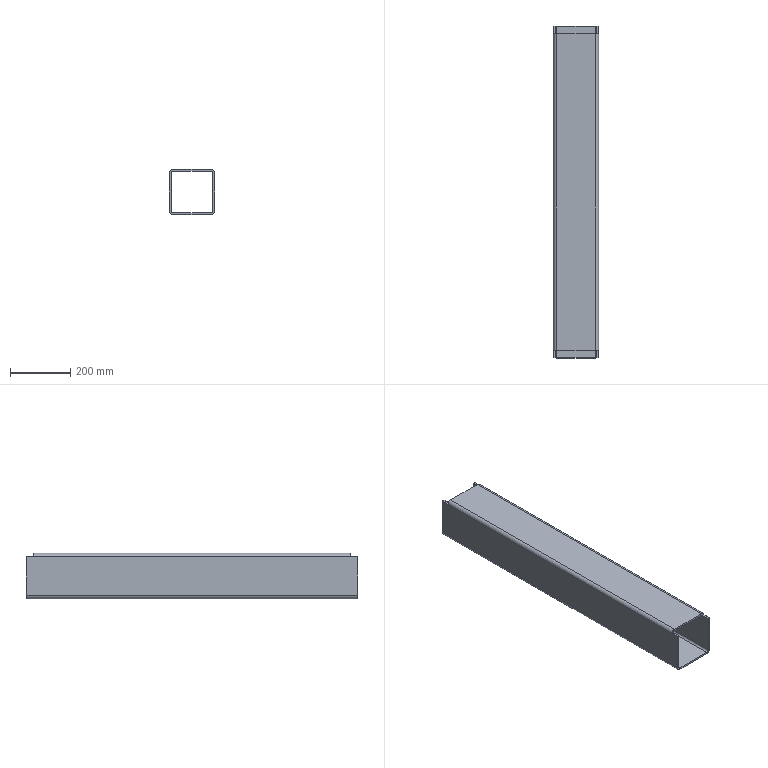Component | SolidWorks | Link1-13 | 1 solid | 24 faces | box 150 x 1100 x 150 mm | volume 3654550 mm3 | plane 16 | cylinder 8 | commonest cylinder face diameters 24 x4 12 x4 | material Plain Carbon Steel
build123d program:
from build123d import *

# Parameters (mm, degrees)
BOSS_EXTRUDE1_DEPTH = 1100
SKETCH3_W           = 150
SKETCH3_H           = 25
CUT_EXTRUDE1_DEPTH  = 10


with BuildPart() as part:
    # Sketch1 → Boss-Extrude1 (new body)
    with BuildSketch(Plane.XY):
        with BuildLine():
            Line((-63, -75), (63, -75))
            ThreePointArc((63, -75), (71.485, -71.485), (75, -63))
            Line((75, -63), (75, 63))
            ThreePointArc((75, 63), (71.485, 71.485), (63, 75))
            Line((63, 75), (-63, 75))
            ThreePointArc((-63, 75), (-71.485, 71.485), (-75, 63))
            Line((-75, 63), (-75, -63))
            ThreePointArc((-75, -63), (-71.485, -71.485), (-63, -75))
        make_face()
        with BuildLine():
            Line((-63, -69), (63, -69))
            ThreePointArc((63, -69), (67.243, -67.243), (69, -63))
            Line((69, -63), (69, 63))
            ThreePointArc((69, 63), (67.243, 67.243), (63, 69))
            Line((63, 69), (-63, 69))
            ThreePointArc((-63, 69), (-67.243, 67.243), (-69, 63))
            Line((-69, 63), (-69, -63))
            ThreePointArc((-69, -63), (-67.243, -67.243), (-63, -69))
        make_face(mode=Mode.SUBTRACT)
    extrude(amount=BOSS_EXTRUDE1_DEPTH)

    # Sketch3 → Cut-Extrude1 (cut)
    with BuildSketch(Plane(origin=(0, 75, 0), x_dir=(1, 0, 0), z_dir=(0, 1, 0))):
        with Locations((0, -12.5)):
            Rectangle(SKETCH3_W, SKETCH3_H)
        with Locations((0, -1087.5)):
            Rectangle(SKETCH3_W, SKETCH3_H)
    extrude(amount=-CUT_EXTRUDE1_DEPTH, mode=Mode.SUBTRACT)


solid = part.part

# Placed as in the assembly
solid = solid.moved(Location((157.801, 1721.323, 5500.973), (90, 0, 0)))
STEP:
#1=COLOUR_RGB('',0.7922,0.8196,0.9333);
#2=FILL_AREA_STYLE_COLOUR('',#1);
#3=FILL_AREA_STYLE('',(#2));
#4=SURFACE_STYLE_FILL_AREA(#3);
#5=SURFACE_SIDE_STYLE('',(#4));
#6=SURFACE_STYLE_USAGE(.BOTH.,#5);
#7=PRESENTATION_STYLE_ASSIGNMENT((#6));
#8=CARTESIAN_POINT('',(3.266,24.462,219.133));
#9=VERTEX_POINT('',#8);
#10=CARTESIAN_POINT('',(3.51,24.462,219.133));
#11=VERTEX_POINT('',#10);
#12=CARTESIAN_POINT('',(9.165,24.462,219.133));
#13=DIRECTION('',(1.,0.,0.));
#14=VECTOR('',#13,39.37);
#15=LINE('',#12,#14);
#16=EDGE_CURVE('',#9,#11,#15,.T.);
#17=ORIENTED_EDGE('',*,*,#16,.F.);
#18=CARTESIAN_POINT('',(3.26,24.462,219.054));
#19=VERTEX_POINT('',#18);
#20=CARTESIAN_POINT('',(3.732,24.462,219.054));
#21=DIRECTION('',(-0.,1.,0.));
#22=DIRECTION('',(-1.,0.,0.));
#23=AXIS2_PLACEMENT_3D('',#20,#21,#22);
#24=CIRCLE('',#23,0.4724);
#25=EDGE_CURVE('',#19,#9,#24,.T.);
#26=ORIENTED_EDGE('',*,*,#25,.F.);
#27=CARTESIAN_POINT('',(3.26,24.462,214.093));
#28=VERTEX_POINT('',#27);
#29=CARTESIAN_POINT('',(3.26,24.462,219.054));
#30=DIRECTION('',(-0.,0.,-1.));
#31=VECTOR('',#30,39.37);
#32=LINE('',#29,#31);
#33=EDGE_CURVE('',#19,#28,#32,.T.);
#34=ORIENTED_EDGE('',*,*,#33,.T.);
#35=CARTESIAN_POINT('',(3.732,24.462,213.621));
#36=VERTEX_POINT('',#35);
#37=CARTESIAN_POINT('',(3.732,24.462,214.093));
#38=DIRECTION('',(-0.,1.,0.));
#39=DIRECTION('',(-1.,0.,0.));
#40=AXIS2_PLACEMENT_3D('',#37,#38,#39);
#41=CIRCLE('',#40,0.4724);
#42=EDGE_CURVE('',#36,#28,#41,.T.);
#43=ORIENTED_EDGE('',*,*,#42,.F.);
#44=CARTESIAN_POINT('',(8.693,24.462,213.621));
#45=VERTEX_POINT('',#44);
#46=CARTESIAN_POINT('',(8.693,24.462,213.621));
#47=DIRECTION('',(-1.,-0.,-0.));
#48=VECTOR('',#47,39.37);
#49=LINE('',#46,#48);
#50=EDGE_CURVE('',#45,#36,#49,.T.);
#51=ORIENTED_EDGE('',*,*,#50,.F.);
#52=CARTESIAN_POINT('',(9.165,24.462,214.093));
#53=VERTEX_POINT('',#52);
#54=CARTESIAN_POINT('',(8.693,24.462,214.093));
#55=DIRECTION('',(-0.,1.,0.));
#56=DIRECTION('',(-1.,0.,0.));
#57=AXIS2_PLACEMENT_3D('',#54,#55,#56);
#58=CIRCLE('',#57,0.4724);
#59=EDGE_CURVE('',#53,#45,#58,.T.);
#60=ORIENTED_EDGE('',*,*,#59,.F.);
#61=CARTESIAN_POINT('',(9.165,24.462,219.054));
#62=VERTEX_POINT('',#61);
#63=CARTESIAN_POINT('',(9.165,24.462,214.093));
#64=DIRECTION('',(0.,-0.,1.));
#65=VECTOR('',#64,39.37);
#66=LINE('',#63,#65);
#67=EDGE_CURVE('',#53,#62,#66,.T.);
#68=ORIENTED_EDGE('',*,*,#67,.T.);
#69=CARTESIAN_POINT('',(9.159,24.462,219.133));
#70=VERTEX_POINT('',#69);
#71=CARTESIAN_POINT('',(8.693,24.462,219.054));
#72=DIRECTION('',(-0.,1.,0.));
#73=DIRECTION('',(-1.,0.,0.));
#74=AXIS2_PLACEMENT_3D('',#71,#72,#73);
#75=CIRCLE('',#74,0.4724);
#76=EDGE_CURVE('',#70,#62,#75,.T.);
#77=ORIENTED_EDGE('',*,*,#76,.F.);
#78=CARTESIAN_POINT('',(8.916,24.462,219.133));
#79=VERTEX_POINT('',#78);
#80=CARTESIAN_POINT('',(9.165,24.462,219.133));
#81=DIRECTION('',(1.,0.,0.));
#82=VECTOR('',#81,39.37);
#83=LINE('',#80,#82);
#84=EDGE_CURVE('',#79,#70,#83,.T.);
#85=ORIENTED_EDGE('',*,*,#84,.F.);
#86=CARTESIAN_POINT('',(8.929,24.462,219.054));
#87=VERTEX_POINT('',#86);
#88=CARTESIAN_POINT('',(8.693,24.462,219.054));
#89=DIRECTION('',(-0.,1.,0.));
#90=DIRECTION('',(-1.,0.,0.));
#91=AXIS2_PLACEMENT_3D('',#88,#89,#90);
#92=CIRCLE('',#91,0.2362);
#93=EDGE_CURVE('',#79,#87,#92,.T.);
#94=ORIENTED_EDGE('',*,*,#93,.T.);
#95=CARTESIAN_POINT('',(8.929,24.462,214.093));
#96=VERTEX_POINT('',#95);
#97=CARTESIAN_POINT('',(8.929,24.462,214.093));
#98=DIRECTION('',(0.,-0.,1.));
#99=VECTOR('',#98,39.37);
#100=LINE('',#97,#99);
#101=EDGE_CURVE('',#96,#87,#100,.T.);
#102=ORIENTED_EDGE('',*,*,#101,.F.);
#103=CARTESIAN_POINT('',(8.693,24.462,213.857));
#104=VERTEX_POINT('',#103);
#105=CARTESIAN_POINT('',(8.693,24.462,214.093));
#106=DIRECTION('',(-0.,1.,0.));
#107=DIRECTION('',(-1.,0.,0.));
#108=AXIS2_PLACEMENT_3D('',#105,#106,#107);
#109=CIRCLE('',#108,0.2362);
#110=EDGE_CURVE('',#96,#104,#109,.T.);
#111=ORIENTED_EDGE('',*,*,#110,.T.);
#112=CARTESIAN_POINT('',(3.732,24.462,213.857));
#113=VERTEX_POINT('',#112);
#114=CARTESIAN_POINT('',(8.693,24.462,213.857));
#115=DIRECTION('',(-1.,-0.,-0.));
#116=VECTOR('',#115,39.37);
#117=LINE('',#114,#116);
#118=EDGE_CURVE('',#104,#113,#117,.T.);
#119=ORIENTED_EDGE('',*,*,#118,.T.);
#120=CARTESIAN_POINT('',(3.496,24.462,214.093));
#121=VERTEX_POINT('',#120);
#122=CARTESIAN_POINT('',(3.732,24.462,214.093));
#123=DIRECTION('',(-0.,1.,0.));
#124=DIRECTION('',(-1.,0.,0.));
#125=AXIS2_PLACEMENT_3D('',#122,#123,#124);
#126=CIRCLE('',#125,0.2362);
#127=EDGE_CURVE('',#113,#121,#126,.T.);
#128=ORIENTED_EDGE('',*,*,#127,.T.);
#129=CARTESIAN_POINT('',(3.496,24.462,219.054));
#130=VERTEX_POINT('',#129);
#131=CARTESIAN_POINT('',(3.496,24.462,219.054));
#132=DIRECTION('',(-0.,0.,-1.));
#133=VECTOR('',#132,39.37);
#134=LINE('',#131,#133);
#135=EDGE_CURVE('',#130,#121,#134,.T.);
#136=ORIENTED_EDGE('',*,*,#135,.F.);
#137=CARTESIAN_POINT('',(3.732,24.462,219.054));
#138=DIRECTION('',(-0.,1.,0.));
#139=DIRECTION('',(-1.,0.,0.));
#140=AXIS2_PLACEMENT_3D('',#137,#138,#139);
#141=CIRCLE('',#140,0.2362);
#142=EDGE_CURVE('',#130,#11,#141,.T.);
#143=ORIENTED_EDGE('',*,*,#142,.T.);
#144=EDGE_LOOP('',(#17,#26,#34,#43,#51,#60,#68,#77,#85,#94,#102,#111,#119,#128,#136,#143));
#145=FACE_OUTER_BOUND('',#144,.T.);
#146=CARTESIAN_POINT('',(3.732,24.462,219.054));
#147=DIRECTION('',(-0.,1.,0.));
#148=DIRECTION('',(-1.,-0.,-0.));
#149=AXIS2_PLACEMENT_3D('',#146,#147,#148);
#150=PLANE('',#149);
#151=ADVANCED_FACE('',(#145),#150,.F.);
#152=CARTESIAN_POINT('',(9.159,67.769,219.133));
#153=VERTEX_POINT('',#152);
#154=CARTESIAN_POINT('',(8.916,67.769,219.133));
#155=VERTEX_POINT('',#154);
#156=CARTESIAN_POINT('',(9.165,67.769,219.133));
#157=DIRECTION('',(-1.,-0.,-0.));
#158=VECTOR('',#157,39.37);
#159=LINE('',#156,#158);
#160=EDGE_CURVE('',#153,#155,#159,.T.);
#161=ORIENTED_EDGE('',*,*,#160,.F.);
#162=CARTESIAN_POINT('',(9.165,67.769,219.054));
#163=VERTEX_POINT('',#162);
#164=CARTESIAN_POINT('',(8.693,67.769,219.054));
#165=DIRECTION('',(-0.,1.,0.));
#166=DIRECTION('',(-1.,0.,0.));
#167=AXIS2_PLACEMENT_3D('',#164,#165,#166);
#168=CIRCLE('',#167,0.4724);
#169=EDGE_CURVE('',#153,#163,#168,.T.);
#170=ORIENTED_EDGE('',*,*,#169,.T.);
#171=CARTESIAN_POINT('',(9.165,67.769,214.093));
#172=VERTEX_POINT('',#171);
#173=CARTESIAN_POINT('',(9.165,67.769,214.093));
#174=DIRECTION('',(0.,-0.,1.));
#175=VECTOR('',#174,39.37);
#176=LINE('',#173,#175);
#177=EDGE_CURVE('',#172,#163,#176,.T.);
#178=ORIENTED_EDGE('',*,*,#177,.F.);
#179=CARTESIAN_POINT('',(8.693,67.769,213.621));
#180=VERTEX_POINT('',#179);
#181=CARTESIAN_POINT('',(8.693,67.769,214.093));
#182=DIRECTION('',(-0.,1.,0.));
#183=DIRECTION('',(-1.,0.,0.));
#184=AXIS2_PLACEMENT_3D('',#181,#182,#183);
#185=CIRCLE('',#184,0.4724);
#186=EDGE_CURVE('',#172,#180,#185,.T.);
#187=ORIENTED_EDGE('',*,*,#186,.T.);
#188=CARTESIAN_POINT('',(3.732,67.769,213.621));
#189=VERTEX_POINT('',#188);
#190=CARTESIAN_POINT('',(8.693,67.769,213.621));
#191=DIRECTION('',(-1.,-0.,-0.));
#192=VECTOR('',#191,39.37);
#193=LINE('',#190,#192);
#194=EDGE_CURVE('',#180,#189,#193,.T.);
#195=ORIENTED_EDGE('',*,*,#194,.T.);
#196=CARTESIAN_POINT('',(3.26,67.769,214.093));
#197=VERTEX_POINT('',#196);
#198=CARTESIAN_POINT('',(3.732,67.769,214.093));
#199=DIRECTION('',(-0.,1.,0.));
#200=DIRECTION('',(-1.,0.,0.));
#201=AXIS2_PLACEMENT_3D('',#198,#199,#200);
#202=CIRCLE('',#201,0.4724);
#203=EDGE_CURVE('',#189,#197,#202,.T.);
#204=ORIENTED_EDGE('',*,*,#203,.T.);
#205=CARTESIAN_POINT('',(3.26,67.769,219.054));
#206=VERTEX_POINT('',#205);
#207=CARTESIAN_POINT('',(3.26,67.769,219.054));
#208=DIRECTION('',(-0.,0.,-1.));
#209=VECTOR('',#208,39.37);
#210=LINE('',#207,#209);
#211=EDGE_CURVE('',#206,#197,#210,.T.);
#212=ORIENTED_EDGE('',*,*,#211,.F.);
#213=CARTESIAN_POINT('',(3.266,67.769,219.133));
#214=VERTEX_POINT('',#213);
#215=CARTESIAN_POINT('',(3.732,67.769,219.054));
#216=DIRECTION('',(-0.,1.,0.));
#217=DIRECTION('',(-1.,0.,0.));
#218=AXIS2_PLACEMENT_3D('',#215,#216,#217);
#219=CIRCLE('',#218,0.4724);
#220=EDGE_CURVE('',#206,#214,#219,.T.);
#221=ORIENTED_EDGE('',*,*,#220,.T.);
#222=CARTESIAN_POINT('',(3.51,67.769,219.133));
#223=VERTEX_POINT('',#222);
#224=CARTESIAN_POINT('',(9.165,67.769,219.133));
#225=DIRECTION('',(-1.,-0.,-0.));
#226=VECTOR('',#225,39.37);
#227=LINE('',#224,#226);
#228=EDGE_CURVE('',#223,#214,#227,.T.);
#229=ORIENTED_EDGE('',*,*,#228,.F.);
#230=CARTESIAN_POINT('',(3.496,67.769,219.054));
#231=VERTEX_POINT('',#230);
#232=CARTESIAN_POINT('',(3.732,67.769,219.054));
#233=DIRECTION('',(-0.,1.,0.));
#234=DIRECTION('',(-1.,0.,0.));
#235=AXIS2_PLACEMENT_3D('',#232,#233,#234);
#236=CIRCLE('',#235,0.2362);
#237=EDGE_CURVE('',#231,#223,#236,.T.);
#238=ORIENTED_EDGE('',*,*,#237,.F.);
#239=CARTESIAN_POINT('',(3.496,67.769,214.093));
#240=VERTEX_POINT('',#239);
#241=CARTESIAN_POINT('',(3.496,67.769,219.054));
#242=DIRECTION('',(-0.,0.,-1.));
#243=VECTOR('',#242,39.37);
#244=LINE('',#241,#243);
#245=EDGE_CURVE('',#231,#240,#244,.T.);
#246=ORIENTED_EDGE('',*,*,#245,.T.);
#247=CARTESIAN_POINT('',(3.732,67.769,213.857));
#248=VERTEX_POINT('',#247);
#249=CARTESIAN_POINT('',(3.732,67.769,214.093));
#250=DIRECTION('',(-0.,1.,0.));
#251=DIRECTION('',(-1.,0.,0.));
#252=AXIS2_PLACEMENT_3D('',#249,#250,#251);
#253=CIRCLE('',#252,0.2362);
#254=EDGE_CURVE('',#248,#240,#253,.T.);
#255=ORIENTED_EDGE('',*,*,#254,.F.);
#256=CARTESIAN_POINT('',(8.693,67.769,213.857));
#257=VERTEX_POINT('',#256);
#258=CARTESIAN_POINT('',(8.693,67.769,213.857));
#259=DIRECTION('',(-1.,-0.,-0.));
#260=VECTOR('',#259,39.37);
#261=LINE('',#258,#260);
#262=EDGE_CURVE('',#257,#248,#261,.T.);
#263=ORIENTED_EDGE('',*,*,#262,.F.);
#264=CARTESIAN_POINT('',(8.929,67.769,214.093));
#265=VERTEX_POINT('',#264);
#266=CARTESIAN_POINT('',(8.693,67.769,214.093));
#267=DIRECTION('',(-0.,1.,0.));
#268=DIRECTION('',(-1.,0.,0.));
#269=AXIS2_PLACEMENT_3D('',#266,#267,#268);
#270=CIRCLE('',#269,0.2362);
#271=EDGE_CURVE('',#265,#257,#270,.T.);
#272=ORIENTED_EDGE('',*,*,#271,.F.);
#273=CARTESIAN_POINT('',(8.929,67.769,219.054));
#274=VERTEX_POINT('',#273);
#275=CARTESIAN_POINT('',(8.929,67.769,214.093));
#276=DIRECTION('',(0.,-0.,1.));
#277=VECTOR('',#276,39.37);
#278=LINE('',#275,#277);
#279=EDGE_CURVE('',#265,#274,#278,.T.);
#280=ORIENTED_EDGE('',*,*,#279,.T.);
#281=CARTESIAN_POINT('',(8.693,67.769,219.054));
#282=DIRECTION('',(-0.,1.,0.));
#283=DIRECTION('',(-1.,0.,0.));
#284=AXIS2_PLACEMENT_3D('',#281,#282,#283);
#285=CIRCLE('',#284,0.2362);
#286=EDGE_CURVE('',#155,#274,#285,.T.);
#287=ORIENTED_EDGE('',*,*,#286,.F.);
#288=EDGE_LOOP('',(#161,#170,#178,#187,#195,#204,#212,#221,#229,#238,#246,#255,#263,#272,#280,#287));
#289=FACE_OUTER_BOUND('',#288,.T.);
#290=CARTESIAN_POINT('',(3.732,67.769,219.054));
#291=DIRECTION('',(-0.,1.,0.));
#292=DIRECTION('',(-1.,-0.,-0.));
#293=AXIS2_PLACEMENT_3D('',#290,#291,#292);
#294=PLANE('',#293);
#295=ADVANCED_FACE('',(#289),#294,.T.);
#296=CARTESIAN_POINT('',(3.266,25.446,219.133));
#297=VERTEX_POINT('',#296);
#298=CARTESIAN_POINT('',(3.266,67.769,219.133));
#299=DIRECTION('',(0.,-1.,-0.));
#300=VECTOR('',#299,39.37);
#301=LINE('',#298,#300);
#302=EDGE_CURVE('',#297,#9,#301,.T.);
#303=ORIENTED_EDGE('',*,*,#302,.F.);
#304=CARTESIAN_POINT('',(3.732,25.446,219.527));
#305=VERTEX_POINT('',#304);
#306=CARTESIAN_POINT('',(3.732,25.446,219.054));
#307=DIRECTION('',(-0.,1.,0.));
#308=DIRECTION('',(-1.,0.,0.));
#309=AXIS2_PLACEMENT_3D('',#306,#307,#308);
#310=CIRCLE('',#309,0.4724);
#311=EDGE_CURVE('',#297,#305,#310,.T.);
#312=ORIENTED_EDGE('',*,*,#311,.T.);
#313=CARTESIAN_POINT('',(3.732,66.784,219.527));
#314=VERTEX_POINT('',#313);
#315=CARTESIAN_POINT('',(3.732,67.769,219.527));
#316=DIRECTION('',(0.,-1.,-0.));
#317=VECTOR('',#316,39.37);
#318=LINE('',#315,#317);
#319=EDGE_CURVE('',#314,#305,#318,.T.);
#320=ORIENTED_EDGE('',*,*,#319,.F.);
#321=CARTESIAN_POINT('',(3.266,66.784,219.133));
#322=VERTEX_POINT('',#321);
#323=CARTESIAN_POINT('',(3.732,66.784,219.054));
#324=DIRECTION('',(0.,-1.,-0.));
#325=DIRECTION('',(1.,0.,0.));
#326=AXIS2_PLACEMENT_3D('',#323,#324,#325);
#327=CIRCLE('',#326,0.4724);
#328=EDGE_CURVE('',#314,#322,#327,.T.);
#329=ORIENTED_EDGE('',*,*,#328,.T.);
#330=CARTESIAN_POINT('',(3.266,67.769,219.133));
#331=DIRECTION('',(-0.,1.,0.));
#332=VECTOR('',#331,39.37);
#333=LINE('',#330,#332);
#334=EDGE_CURVE('',#322,#214,#333,.T.);
#335=ORIENTED_EDGE('',*,*,#334,.T.);
#336=ORIENTED_EDGE('',*,*,#220,.F.);
#337=CARTESIAN_POINT('',(3.26,67.769,219.054));
#338=DIRECTION('',(0.,-1.,-0.));
#339=VECTOR('',#338,39.37);
#340=LINE('',#337,#339);
#341=EDGE_CURVE('',#206,#19,#340,.T.);
#342=ORIENTED_EDGE('',*,*,#341,.T.);
#343=ORIENTED_EDGE('',*,*,#25,.T.);
#344=EDGE_LOOP('',(#303,#312,#320,#329,#335,#336,#342,#343));
#345=FACE_OUTER_BOUND('',#344,.T.);
#346=CARTESIAN_POINT('',(3.732,67.769,219.054));
#347=DIRECTION('',(0.,-1.,-0.));
#348=DIRECTION('',(1.,0.,0.));
#349=AXIS2_PLACEMENT_3D('',#346,#347,#348);
#350=CYLINDRICAL_SURFACE('',#349,0.4724);
#351=ADVANCED_FACE('',(#345),#350,.T.);
#352=ORIENTED_EDGE('',*,*,#319,.T.);
#353=CARTESIAN_POINT('',(8.693,25.446,219.527));
#354=VERTEX_POINT('',#353);
#355=CARTESIAN_POINT('',(9.165,25.446,219.527));
#356=DIRECTION('',(-1.,-0.,-0.));
#357=VECTOR('',#356,39.37);
#358=LINE('',#355,#357);
#359=EDGE_CURVE('',#354,#305,#358,.T.);
#360=ORIENTED_EDGE('',*,*,#359,.F.);
#361=CARTESIAN_POINT('',(8.693,66.784,219.527));
#362=VERTEX_POINT('',#361);
#363=CARTESIAN_POINT('',(8.693,67.769,219.527));
#364=DIRECTION('',(0.,-1.,-0.));
#365=VECTOR('',#364,39.37);
#366=LINE('',#363,#365);
#367=EDGE_CURVE('',#362,#354,#366,.T.);
#368=ORIENTED_EDGE('',*,*,#367,.F.);
#369=CARTESIAN_POINT('',(9.165,66.784,219.527));
#370=DIRECTION('',(1.,0.,0.));
#371=VECTOR('',#370,39.37);
#372=LINE('',#369,#371);
#373=EDGE_CURVE('',#314,#362,#372,.T.);
#374=ORIENTED_EDGE('',*,*,#373,.F.);
#375=EDGE_LOOP('',(#352,#360,#368,#374));
#376=FACE_OUTER_BOUND('',#375,.T.);
#377=CARTESIAN_POINT('',(3.732,67.769,219.527));
#378=DIRECTION('',(-0.,0.,-1.));
#379=DIRECTION('',(0.,-1.,-0.));
#380=AXIS2_PLACEMENT_3D('',#377,#378,#379);
#381=PLANE('',#380);
#382=ADVANCED_FACE('',(#376),#381,.F.);
#383=ORIENTED_EDGE('',*,*,#367,.T.);
#384=CARTESIAN_POINT('',(9.159,25.446,219.133));
#385=VERTEX_POINT('',#384);
#386=CARTESIAN_POINT('',(8.693,25.446,219.054));
#387=DIRECTION('',(-0.,1.,0.));
#388=DIRECTION('',(-1.,0.,0.));
#389=AXIS2_PLACEMENT_3D('',#386,#387,#388);
#390=CIRCLE('',#389,0.4724);
#391=EDGE_CURVE('',#354,#385,#390,.T.);
#392=ORIENTED_EDGE('',*,*,#391,.T.);
#393=CARTESIAN_POINT('',(9.159,67.769,219.133));
#394=DIRECTION('',(-0.,1.,0.));
#395=VECTOR('',#394,39.37);
#396=LINE('',#393,#395);
#397=EDGE_CURVE('',#70,#385,#396,.T.);
#398=ORIENTED_EDGE('',*,*,#397,.F.);
#399=ORIENTED_EDGE('',*,*,#76,.T.);
#400=CARTESIAN_POINT('',(9.165,67.769,219.054));
#401=DIRECTION('',(0.,-1.,-0.));
#402=VECTOR('',#401,39.37);
#403=LINE('',#400,#402);
#404=EDGE_CURVE('',#163,#62,#403,.T.);
#405=ORIENTED_EDGE('',*,*,#404,.F.);
#406=ORIENTED_EDGE('',*,*,#169,.F.);
#407=CARTESIAN_POINT('',(9.159,66.784,219.133));
#408=VERTEX_POINT('',#407);
#409=CARTESIAN_POINT('',(9.159,67.769,219.133));
#410=DIRECTION('',(0.,-1.,-0.));
#411=VECTOR('',#410,39.37);
#412=LINE('',#409,#411);
#413=EDGE_CURVE('',#153,#408,#412,.T.);
#414=ORIENTED_EDGE('',*,*,#413,.T.);
#415=CARTESIAN_POINT('',(8.693,66.784,219.054));
#416=DIRECTION('',(0.,-1.,-0.));
#417=DIRECTION('',(1.,0.,0.));
#418=AXIS2_PLACEMENT_3D('',#415,#416,#417);
#419=CIRCLE('',#418,0.4724);
#420=EDGE_CURVE('',#408,#362,#419,.T.);
#421=ORIENTED_EDGE('',*,*,#420,.T.);
#422=EDGE_LOOP('',(#383,#392,#398,#399,#405,#406,#414,#421));
#423=FACE_OUTER_BOUND('',#422,.T.);
#424=CARTESIAN_POINT('',(8.693,67.769,219.054));
#425=DIRECTION('',(0.,-1.,-0.));
#426=DIRECTION('',(1.,0.,0.));
#427=AXIS2_PLACEMENT_3D('',#424,#425,#426);
#428=CYLINDRICAL_SURFACE('',#427,0.4724);
#429=ADVANCED_FACE('',(#423),#428,.T.);
#430=ORIENTED_EDGE('',*,*,#67,.F.);
#431=CARTESIAN_POINT('',(9.165,67.769,214.093));
#432=DIRECTION('',(0.,-1.,-0.));
#433=VECTOR('',#432,39.37);
#434=LINE('',#431,#433);
#435=EDGE_CURVE('',#172,#53,#434,.T.);
#436=ORIENTED_EDGE('',*,*,#435,.F.);
#437=ORIENTED_EDGE('',*,*,#177,.T.);
#438=ORIENTED_EDGE('',*,*,#404,.T.);
#439=EDGE_LOOP('',(#430,#436,#437,#438));
#440=FACE_OUTER_BOUND('',#439,.T.);
#441=CARTESIAN_POINT('',(9.165,67.769,214.093));
#442=DIRECTION('',(1.,0.,0.));
#443=DIRECTION('',(-0.,1.,0.));
#444=AXIS2_PLACEMENT_3D('',#441,#442,#443);
#445=PLANE('',#444);
#446=ADVANCED_FACE('',(#440),#445,.T.);
#447=ORIENTED_EDGE('',*,*,#59,.T.);
#448=CARTESIAN_POINT('',(8.693,67.769,213.621));
#449=DIRECTION('',(0.,-1.,-0.));
#450=VECTOR('',#449,39.37);
#451=LINE('',#448,#450);
#452=EDGE_CURVE('',#180,#45,#451,.T.);
#453=ORIENTED_EDGE('',*,*,#452,.F.);
#454=ORIENTED_EDGE('',*,*,#186,.F.);
#455=ORIENTED_EDGE('',*,*,#435,.T.);
#456=EDGE_LOOP('',(#447,#453,#454,#455));
#457=FACE_OUTER_BOUND('',#456,.T.);
#458=CARTESIAN_POINT('',(8.693,67.769,214.093));
#459=DIRECTION('',(0.,-1.,-0.));
#460=DIRECTION('',(1.,0.,0.));
#461=AXIS2_PLACEMENT_3D('',#458,#459,#460);
#462=CYLINDRICAL_SURFACE('',#461,0.4724);
#463=ADVANCED_FACE('',(#457),#462,.T.);
#464=ORIENTED_EDGE('',*,*,#50,.T.);
#465=CARTESIAN_POINT('',(3.732,67.769,213.621));
#466=DIRECTION('',(0.,-1.,-0.));
#467=VECTOR('',#466,39.37);
#468=LINE('',#465,#467);
#469=EDGE_CURVE('',#189,#36,#468,.T.);
#470=ORIENTED_EDGE('',*,*,#469,.F.);
#471=ORIENTED_EDGE('',*,*,#194,.F.);
#472=ORIENTED_EDGE('',*,*,#452,.T.);
#473=EDGE_LOOP('',(#464,#470,#471,#472));
#474=FACE_OUTER_BOUND('',#473,.T.);
#475=CARTESIAN_POINT('',(8.693,67.769,213.621));
#476=DIRECTION('',(0.,-0.,1.));
#477=DIRECTION('',(-0.,1.,0.));
#478=AXIS2_PLACEMENT_3D('',#475,#476,#477);
#479=PLANE('',#478);
#480=ADVANCED_FACE('',(#474),#479,.F.);
#481=ORIENTED_EDGE('',*,*,#42,.T.);
#482=CARTESIAN_POINT('',(3.26,67.769,214.093));
#483=DIRECTION('',(0.,-1.,-0.));
#484=VECTOR('',#483,39.37);
#485=LINE('',#482,#484);
#486=EDGE_CURVE('',#197,#28,#485,.T.);
#487=ORIENTED_EDGE('',*,*,#486,.F.);
#488=ORIENTED_EDGE('',*,*,#203,.F.);
#489=ORIENTED_EDGE('',*,*,#469,.T.);
#490=EDGE_LOOP('',(#481,#487,#488,#489));
#491=FACE_OUTER_BOUND('',#490,.T.);
#492=CARTESIAN_POINT('',(3.732,67.769,214.093));
#493=DIRECTION('',(0.,-1.,-0.));
#494=DIRECTION('',(1.,0.,0.));
#495=AXIS2_PLACEMENT_3D('',#492,#493,#494);
#496=CYLINDRICAL_SURFACE('',#495,0.4724);
#497=ADVANCED_FACE('',(#491),#496,.T.);
#498=ORIENTED_EDGE('',*,*,#33,.F.);
#499=ORIENTED_EDGE('',*,*,#341,.F.);
#500=ORIENTED_EDGE('',*,*,#211,.T.);
#501=ORIENTED_EDGE('',*,*,#486,.T.);
#502=EDGE_LOOP('',(#498,#499,#500,#501));
#503=FACE_OUTER_BOUND('',#502,.T.);
#504=CARTESIAN_POINT('',(3.26,67.769,219.054));
#505=DIRECTION('',(-1.,-0.,-0.));
#506=DIRECTION('',(0.,-1.,-0.));
#507=AXIS2_PLACEMENT_3D('',#504,#505,#506);
#508=PLANE('',#507);
#509=ADVANCED_FACE('',(#503),#508,.T.);
#510=ORIENTED_EDGE('',*,*,#110,.F.);
#511=CARTESIAN_POINT('',(8.929,67.769,214.093));
#512=DIRECTION('',(0.,-1.,-0.));
#513=VECTOR('',#512,39.37);
#514=LINE('',#511,#513);
#515=EDGE_CURVE('',#265,#96,#514,.T.);
#516=ORIENTED_EDGE('',*,*,#515,.F.);
#517=ORIENTED_EDGE('',*,*,#271,.T.);
#518=CARTESIAN_POINT('',(8.693,67.769,213.857));
#519=DIRECTION('',(0.,-1.,-0.));
#520=VECTOR('',#519,39.37);
#521=LINE('',#518,#520);
#522=EDGE_CURVE('',#257,#104,#521,.T.);
#523=ORIENTED_EDGE('',*,*,#522,.T.);
#524=EDGE_LOOP('',(#510,#516,#517,#523));
#525=FACE_OUTER_BOUND('',#524,.T.);
#526=CARTESIAN_POINT('',(8.693,67.769,214.093));
#527=DIRECTION('',(0.,-1.,-0.));
#528=DIRECTION('',(1.,0.,0.));
#529=AXIS2_PLACEMENT_3D('',#526,#527,#528);
#530=CYLINDRICAL_SURFACE('',#529,0.2362);
#531=ADVANCED_FACE('',(#525),#530,.F.);
#532=ORIENTED_EDGE('',*,*,#118,.F.);
#533=ORIENTED_EDGE('',*,*,#522,.F.);
#534=ORIENTED_EDGE('',*,*,#262,.T.);
#535=CARTESIAN_POINT('',(3.732,67.769,213.857));
#536=DIRECTION('',(0.,-1.,-0.));
#537=VECTOR('',#536,39.37);
#538=LINE('',#535,#537);
#539=EDGE_CURVE('',#248,#113,#538,.T.);
#540=ORIENTED_EDGE('',*,*,#539,.T.);
#541=EDGE_LOOP('',(#532,#533,#534,#540));
#542=FACE_OUTER_BOUND('',#541,.T.);
#543=CARTESIAN_POINT('',(8.693,67.769,213.857));
#544=DIRECTION('',(0.,-0.,1.));
#545=DIRECTION('',(-0.,1.,0.));
#546=AXIS2_PLACEMENT_3D('',#543,#544,#545);
#547=PLANE('',#546);
#548=ADVANCED_FACE('',(#542),#547,.T.);
#549=ORIENTED_EDGE('',*,*,#127,.F.);
#550=ORIENTED_EDGE('',*,*,#539,.F.);
#551=ORIENTED_EDGE('',*,*,#254,.T.);
#552=CARTESIAN_POINT('',(3.496,67.769,214.093));
#553=DIRECTION('',(0.,-1.,-0.));
#554=VECTOR('',#553,39.37);
#555=LINE('',#552,#554);
#556=EDGE_CURVE('',#240,#121,#555,.T.);
#557=ORIENTED_EDGE('',*,*,#556,.T.);
#558=EDGE_LOOP('',(#549,#550,#551,#557));
#559=FACE_OUTER_BOUND('',#558,.T.);
#560=CARTESIAN_POINT('',(3.732,67.769,214.093));
#561=DIRECTION('',(0.,-1.,-0.));
#562=DIRECTION('',(1.,0.,0.));
#563=AXIS2_PLACEMENT_3D('',#560,#561,#562);
#564=CYLINDRICAL_SURFACE('',#563,0.2362);
#565=ADVANCED_FACE('',(#559),#564,.F.);
#566=ORIENTED_EDGE('',*,*,#135,.T.);
#567=ORIENTED_EDGE('',*,*,#556,.F.);
#568=ORIENTED_EDGE('',*,*,#245,.F.);
#569=CARTESIAN_POINT('',(3.496,67.769,219.054));
#570=DIRECTION('',(0.,-1.,-0.));
#571=VECTOR('',#570,39.37);
#572=LINE('',#569,#571);
#573=EDGE_CURVE('',#231,#130,#572,.T.);
#574=ORIENTED_EDGE('',*,*,#573,.T.);
#575=EDGE_LOOP('',(#566,#567,#568,#574));
#576=FACE_OUTER_BOUND('',#575,.T.);
#577=CARTESIAN_POINT('',(3.496,67.769,219.054));
#578=DIRECTION('',(-1.,-0.,-0.));
#579=DIRECTION('',(0.,-1.,-0.));
#580=AXIS2_PLACEMENT_3D('',#577,#578,#579);
#581=PLANE('',#580);
#582=ADVANCED_FACE('',(#576),#581,.F.);
#583=CARTESIAN_POINT('',(3.51,25.446,219.133));
#584=VERTEX_POINT('',#583);
#585=CARTESIAN_POINT('',(3.732,25.446,219.29));
#586=VERTEX_POINT('',#585);
#587=CARTESIAN_POINT('',(3.732,25.446,219.054));
#588=DIRECTION('',(-0.,1.,0.));
#589=DIRECTION('',(-1.,0.,0.));
#590=AXIS2_PLACEMENT_3D('',#587,#588,#589);
#591=CIRCLE('',#590,0.2362);
#592=EDGE_CURVE('',#584,#586,#591,.T.);
#593=ORIENTED_EDGE('',*,*,#592,.F.);
#594=CARTESIAN_POINT('',(3.51,67.769,219.133));
#595=DIRECTION('',(0.,-1.,-0.));
#596=VECTOR('',#595,39.37);
#597=LINE('',#594,#596);
#598=EDGE_CURVE('',#584,#11,#597,.T.);
#599=ORIENTED_EDGE('',*,*,#598,.T.);
#600=ORIENTED_EDGE('',*,*,#142,.F.);
#601=ORIENTED_EDGE('',*,*,#573,.F.);
#602=ORIENTED_EDGE('',*,*,#237,.T.);
#603=CARTESIAN_POINT('',(3.51,66.784,219.133));
#604=VERTEX_POINT('',#603);
#605=CARTESIAN_POINT('',(3.51,67.769,219.133));
#606=DIRECTION('',(-0.,1.,0.));
#607=VECTOR('',#606,39.37);
#608=LINE('',#605,#607);
#609=EDGE_CURVE('',#604,#223,#608,.T.);
#610=ORIENTED_EDGE('',*,*,#609,.F.);
#611=CARTESIAN_POINT('',(3.732,66.784,219.29));
#612=VERTEX_POINT('',#611);
#613=CARTESIAN_POINT('',(3.732,66.784,219.054));
#614=DIRECTION('',(0.,-1.,-0.));
#615=DIRECTION('',(1.,0.,0.));
#616=AXIS2_PLACEMENT_3D('',#613,#614,#615);
#617=CIRCLE('',#616,0.2362);
#618=EDGE_CURVE('',#612,#604,#617,.T.);
#619=ORIENTED_EDGE('',*,*,#618,.F.);
#620=CARTESIAN_POINT('',(3.732,67.769,219.29));
#621=DIRECTION('',(0.,-1.,-0.));
#622=VECTOR('',#621,39.37);
#623=LINE('',#620,#622);
#624=EDGE_CURVE('',#612,#586,#623,.T.);
#625=ORIENTED_EDGE('',*,*,#624,.T.);
#626=EDGE_LOOP('',(#593,#599,#600,#601,#602,#610,#619,#625));
#627=FACE_OUTER_BOUND('',#626,.T.);
#628=CARTESIAN_POINT('',(3.732,67.769,219.054));
#629=DIRECTION('',(0.,-1.,-0.));
#630=DIRECTION('',(1.,0.,0.));
#631=AXIS2_PLACEMENT_3D('',#628,#629,#630);
#632=CYLINDRICAL_SURFACE('',#631,0.2362);
#633=ADVANCED_FACE('',(#627),#632,.F.);
#634=CARTESIAN_POINT('',(8.693,25.446,219.29));
#635=VERTEX_POINT('',#634);
#636=CARTESIAN_POINT('',(3.732,25.446,219.29));
#637=DIRECTION('',(1.,0.,0.));
#638=VECTOR('',#637,39.37);
#639=LINE('',#636,#638);
#640=EDGE_CURVE('',#586,#635,#639,.T.);
#641=ORIENTED_EDGE('',*,*,#640,.F.);
#642=ORIENTED_EDGE('',*,*,#624,.F.);
#643=CARTESIAN_POINT('',(8.693,66.784,219.29));
#644=VERTEX_POINT('',#643);
#645=CARTESIAN_POINT('',(3.732,66.784,219.29));
#646=DIRECTION('',(-1.,-0.,-0.));
#647=VECTOR('',#646,39.37);
#648=LINE('',#645,#647);
#649=EDGE_CURVE('',#644,#612,#648,.T.);
#650=ORIENTED_EDGE('',*,*,#649,.F.);
#651=CARTESIAN_POINT('',(8.693,67.769,219.29));
#652=DIRECTION('',(0.,-1.,-0.));
#653=VECTOR('',#652,39.37);
#654=LINE('',#651,#653);
#655=EDGE_CURVE('',#644,#635,#654,.T.);
#656=ORIENTED_EDGE('',*,*,#655,.T.);
#657=EDGE_LOOP('',(#641,#642,#650,#656));
#658=FACE_OUTER_BOUND('',#657,.T.);
#659=CARTESIAN_POINT('',(3.732,67.769,219.29));
#660=DIRECTION('',(-0.,0.,-1.));
#661=DIRECTION('',(0.,-1.,-0.));
#662=AXIS2_PLACEMENT_3D('',#659,#660,#661);
#663=PLANE('',#662);
#664=ADVANCED_FACE('',(#658),#663,.T.);
#665=CARTESIAN_POINT('',(8.916,25.446,219.133));
#666=VERTEX_POINT('',#665);
#667=CARTESIAN_POINT('',(8.693,25.446,219.054));
#668=DIRECTION('',(-0.,1.,0.));
#669=DIRECTION('',(-1.,0.,0.));
#670=AXIS2_PLACEMENT_3D('',#667,#668,#669);
#671=CIRCLE('',#670,0.2362);
#672=EDGE_CURVE('',#635,#666,#671,.T.);
#673=ORIENTED_EDGE('',*,*,#672,.F.);
#674=ORIENTED_EDGE('',*,*,#655,.F.);
#675=CARTESIAN_POINT('',(8.916,66.784,219.133));
#676=VERTEX_POINT('',#675);
#677=CARTESIAN_POINT('',(8.693,66.784,219.054));
#678=DIRECTION('',(0.,-1.,-0.));
#679=DIRECTION('',(1.,0.,0.));
#680=AXIS2_PLACEMENT_3D('',#677,#678,#679);
#681=CIRCLE('',#680,0.2362);
#682=EDGE_CURVE('',#676,#644,#681,.T.);
#683=ORIENTED_EDGE('',*,*,#682,.F.);
#684=CARTESIAN_POINT('',(8.916,67.769,219.133));
#685=DIRECTION('',(0.,-1.,-0.));
#686=VECTOR('',#685,39.37);
#687=LINE('',#684,#686);
#688=EDGE_CURVE('',#155,#676,#687,.T.);
#689=ORIENTED_EDGE('',*,*,#688,.F.);
#690=ORIENTED_EDGE('',*,*,#286,.T.);
#691=CARTESIAN_POINT('',(8.929,67.769,219.054));
#692=DIRECTION('',(0.,-1.,-0.));
#693=VECTOR('',#692,39.37);
#694=LINE('',#691,#693);
#695=EDGE_CURVE('',#274,#87,#694,.T.);
#696=ORIENTED_EDGE('',*,*,#695,.T.);
#697=ORIENTED_EDGE('',*,*,#93,.F.);
#698=CARTESIAN_POINT('',(8.916,67.769,219.133));
#699=DIRECTION('',(-0.,1.,0.));
#700=VECTOR('',#699,39.37);
#701=LINE('',#698,#700);
#702=EDGE_CURVE('',#79,#666,#701,.T.);
#703=ORIENTED_EDGE('',*,*,#702,.T.);
#704=EDGE_LOOP('',(#673,#674,#683,#689,#690,#696,#697,#703));
#705=FACE_OUTER_BOUND('',#704,.T.);
#706=CARTESIAN_POINT('',(8.693,67.769,219.054));
#707=DIRECTION('',(0.,-1.,-0.));
#708=DIRECTION('',(1.,0.,0.));
#709=AXIS2_PLACEMENT_3D('',#706,#707,#708);
#710=CYLINDRICAL_SURFACE('',#709,0.2362);
#711=ADVANCED_FACE('',(#705),#710,.F.);
#712=ORIENTED_EDGE('',*,*,#101,.T.);
#713=ORIENTED_EDGE('',*,*,#695,.F.);
#714=ORIENTED_EDGE('',*,*,#279,.F.);
#715=ORIENTED_EDGE('',*,*,#515,.T.);
#716=EDGE_LOOP('',(#712,#713,#714,#715));
#717=FACE_OUTER_BOUND('',#716,.T.);
#718=CARTESIAN_POINT('',(8.929,67.769,214.093));
#719=DIRECTION('',(1.,0.,0.));
#720=DIRECTION('',(-0.,1.,0.));
#721=AXIS2_PLACEMENT_3D('',#718,#719,#720);
#722=PLANE('',#721);
#723=ADVANCED_FACE('',(#717),#722,.F.);
#724=ORIENTED_EDGE('',*,*,#373,.T.);
#725=ORIENTED_EDGE('',*,*,#420,.F.);
#726=CARTESIAN_POINT('',(9.165,66.784,219.133));
#727=DIRECTION('',(1.,0.,0.));
#728=VECTOR('',#727,39.37);
#729=LINE('',#726,#728);
#730=EDGE_CURVE('',#676,#408,#729,.T.);
#731=ORIENTED_EDGE('',*,*,#730,.F.);
#732=ORIENTED_EDGE('',*,*,#682,.T.);
#733=ORIENTED_EDGE('',*,*,#649,.T.);
#734=ORIENTED_EDGE('',*,*,#618,.T.);
#735=CARTESIAN_POINT('',(9.165,66.784,219.133));
#736=DIRECTION('',(1.,0.,0.));
#737=VECTOR('',#736,39.37);
#738=LINE('',#735,#737);
#739=EDGE_CURVE('',#322,#604,#738,.T.);
#740=ORIENTED_EDGE('',*,*,#739,.F.);
#741=ORIENTED_EDGE('',*,*,#328,.F.);
#742=EDGE_LOOP('',(#724,#725,#731,#732,#733,#734,#740,#741));
#743=FACE_OUTER_BOUND('',#742,.T.);
#744=CARTESIAN_POINT('',(9.165,66.784,219.133));
#745=DIRECTION('',(0.,-1.,-0.));
#746=DIRECTION('',(1.,0.,0.));
#747=AXIS2_PLACEMENT_3D('',#744,#745,#746);
#748=PLANE('',#747);
#749=ADVANCED_FACE('',(#743),#748,.F.);
#750=ORIENTED_EDGE('',*,*,#739,.T.);
#751=ORIENTED_EDGE('',*,*,#609,.T.);
#752=ORIENTED_EDGE('',*,*,#228,.T.);
#753=ORIENTED_EDGE('',*,*,#334,.F.);
#754=EDGE_LOOP('',(#750,#751,#752,#753));
#755=FACE_OUTER_BOUND('',#754,.T.);
#756=CARTESIAN_POINT('',(6.213,24.462,219.133));
#757=DIRECTION('',(-0.,0.,-1.));
#758=DIRECTION('',(0.,-1.,-0.));
#759=AXIS2_PLACEMENT_3D('',#756,#757,#758);
#760=PLANE('',#759);
#761=ADVANCED_FACE('',(#755),#760,.F.);
#762=ORIENTED_EDGE('',*,*,#160,.T.);
#763=ORIENTED_EDGE('',*,*,#688,.T.);
#764=ORIENTED_EDGE('',*,*,#730,.T.);
#765=ORIENTED_EDGE('',*,*,#413,.F.);
#766=EDGE_LOOP('',(#762,#763,#764,#765));
#767=FACE_OUTER_BOUND('',#766,.T.);
#768=CARTESIAN_POINT('',(6.213,24.462,219.133));
#769=DIRECTION('',(-0.,0.,-1.));
#770=DIRECTION('',(0.,-1.,-0.));
#771=AXIS2_PLACEMENT_3D('',#768,#769,#770);
#772=PLANE('',#771);
#773=ADVANCED_FACE('',(#767),#772,.F.);
#774=CARTESIAN_POINT('',(9.165,25.446,219.133));
#775=DIRECTION('',(-1.,-0.,-0.));
#776=VECTOR('',#775,39.37);
#777=LINE('',#774,#776);
#778=EDGE_CURVE('',#584,#297,#777,.T.);
#779=ORIENTED_EDGE('',*,*,#778,.F.);
#780=ORIENTED_EDGE('',*,*,#592,.T.);
#781=ORIENTED_EDGE('',*,*,#640,.T.);
#782=ORIENTED_EDGE('',*,*,#672,.T.);
#783=CARTESIAN_POINT('',(9.165,25.446,219.133));
#784=DIRECTION('',(-1.,-0.,-0.));
#785=VECTOR('',#784,39.37);
#786=LINE('',#783,#785);
#787=EDGE_CURVE('',#385,#666,#786,.T.);
#788=ORIENTED_EDGE('',*,*,#787,.F.);
#789=ORIENTED_EDGE('',*,*,#391,.F.);
#790=ORIENTED_EDGE('',*,*,#359,.T.);
#791=ORIENTED_EDGE('',*,*,#311,.F.);
#792=EDGE_LOOP('',(#779,#780,#781,#782,#788,#789,#790,#791));
#793=FACE_OUTER_BOUND('',#792,.T.);
#794=CARTESIAN_POINT('',(9.165,25.446,219.133));
#795=DIRECTION('',(-0.,1.,0.));
#796=DIRECTION('',(-1.,-0.,-0.));
#797=AXIS2_PLACEMENT_3D('',#794,#795,#796);
#798=PLANE('',#797);
#799=ADVANCED_FACE('',(#793),#798,.F.);
#800=ORIENTED_EDGE('',*,*,#302,.T.);
#801=ORIENTED_EDGE('',*,*,#16,.T.);
#802=ORIENTED_EDGE('',*,*,#598,.F.);
#803=ORIENTED_EDGE('',*,*,#778,.T.);
#804=EDGE_LOOP('',(#800,#801,#802,#803));
#805=FACE_OUTER_BOUND('',#804,.T.);
#806=CARTESIAN_POINT('',(6.213,24.462,219.133));
#807=DIRECTION('',(0.,-0.,1.));
#808=DIRECTION('',(-0.,1.,0.));
#809=AXIS2_PLACEMENT_3D('',#806,#807,#808);
#810=PLANE('',#809);
#811=ADVANCED_FACE('',(#805),#810,.T.);
#812=ORIENTED_EDGE('',*,*,#397,.T.);
#813=ORIENTED_EDGE('',*,*,#787,.T.);
#814=ORIENTED_EDGE('',*,*,#702,.F.);
#815=ORIENTED_EDGE('',*,*,#84,.T.);
#816=EDGE_LOOP('',(#812,#813,#814,#815));
#817=FACE_OUTER_BOUND('',#816,.T.);
#818=CARTESIAN_POINT('',(6.213,24.462,219.133));
#819=DIRECTION('',(0.,-0.,1.));
#820=DIRECTION('',(-0.,1.,0.));
#821=AXIS2_PLACEMENT_3D('',#818,#819,#820);
#822=PLANE('',#821);
#823=ADVANCED_FACE('',(#817),#822,.T.);
#824=CLOSED_SHELL('',(#151,#295,#351,#382,#429,#446,#463,#480,#497,#509,#531,#548,#565,#582,#633,#664,#711,#723,#749,#761,#773,#799,#811,#823));
#825=MANIFOLD_SOLID_BREP('',#824);
#826=STYLED_ITEM('',(#7),#825);
#827=(LENGTH_UNIT()NAMED_UNIT(*)SI_UNIT($,.METRE.));
#828=LENGTH_MEASURE_WITH_UNIT(LENGTH_MEASURE(0.0254),#827);
#829=DIMENSIONAL_EXPONENTS(1.,0.,0.,0.,0.,0.,0.);
#830=(CONVERSION_BASED_UNIT('',#828)LENGTH_UNIT()NAMED_UNIT(#829));
#831=UNCERTAINTY_MEASURE_WITH_UNIT(LENGTH_MEASURE(0.00001),#830,'','');
#832=(NAMED_UNIT(*)PLANE_ANGLE_UNIT()SI_UNIT($,.RADIAN.));
#833=(NAMED_UNIT(*)SI_UNIT($,.STERADIAN.)SOLID_ANGLE_UNIT());
#834=(GEOMETRIC_REPRESENTATION_CONTEXT(3)GLOBAL_UNCERTAINTY_ASSIGNED_CONTEXT((#831))GLOBAL_UNIT_ASSIGNED_CONTEXT((#830,#832,#833))REPRESENTATION_CONTEXT('',''));
#835=MECHANICAL_DESIGN_GEOMETRIC_PRESENTATION_REPRESENTATION('',(#826),#834);
#836=PRESENTATION_LAYER_ASSIGNMENT('','',(#826));
#837=CARTESIAN_POINT('',(0.,0.,0.));
#838=DIRECTION('',(0.,0.,1.));
#839=DIRECTION('',(1.,0.,0.));
#840=AXIS2_PLACEMENT_3D('',#837,#838,#839);
#841=(LENGTH_UNIT()NAMED_UNIT(*)SI_UNIT($,.METRE.));
#842=LENGTH_MEASURE_WITH_UNIT(LENGTH_MEASURE(0.0254),#841);
#843=DIMENSIONAL_EXPONENTS(1.,0.,0.,0.,0.,0.,0.);
#844=(CONVERSION_BASED_UNIT('',#842)LENGTH_UNIT()NAMED_UNIT(#843));
#845=UNCERTAINTY_MEASURE_WITH_UNIT(LENGTH_MEASURE(0.00001),#844,'','');
#846=(NAMED_UNIT(*)PLANE_ANGLE_UNIT()SI_UNIT($,.RADIAN.));
#847=(NAMED_UNIT(*)SI_UNIT($,.STERADIAN.)SOLID_ANGLE_UNIT());
#848=(GEOMETRIC_REPRESENTATION_CONTEXT(3)GLOBAL_UNCERTAINTY_ASSIGNED_CONTEXT((#845))GLOBAL_UNIT_ASSIGNED_CONTEXT((#844,#846,#847))REPRESENTATION_CONTEXT('',''));
#849=ADVANCED_BREP_SHAPE_REPRESENTATION('',(#825,#840),#848);